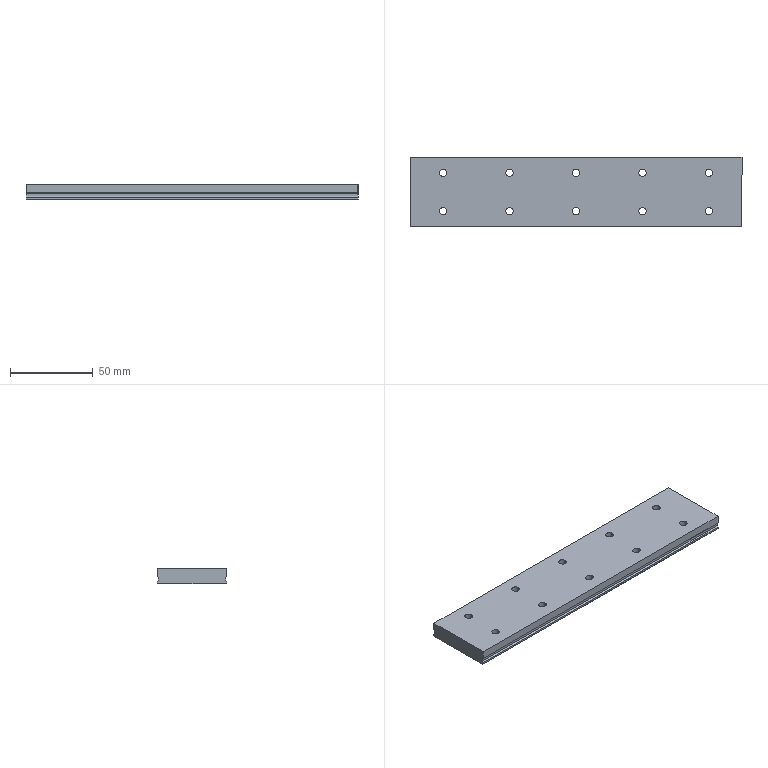Component | SolidWorks | SRS15WM-240GuideRail-2-2 | 1 solid | 66 faces | box 200 x 42 x 9.5 mm | volume 76129 mm3 | cylinder 40 | plane 26 | commonest cylinder face diameters 4.5 x20 8 x20
build123d program:
from build123d import *

# Parameters (mm, degrees)
BOSS_EXTRUDE1_DEPTH                                 = 200
CHAMFER1_SIZE                                       = 0.5
M4_COUNTERSUNK_HOLE_FOR_SOCKET_HEAD_CAP_D           = 4.5
M4_COUNTERSUNK_HOLE_FOR_SOCKET_HEAD_CAP_CBORE_D     = 8
M4_COUNTERSUNK_HOLE_FOR_SOCKET_HEAD_CAP_CBORE_DEPTH = 4
LPATTERN1_COUNT                                     = 5
LPATTERN1_PITCH                                     = 40


with BuildPart() as part:
    # Sketch1 → Boss-Extrude1 (new body)
    with BuildSketch(Plane.XY):
        Polygon((0, 8), (0.8, 7.2), (0.8, 5.7), (0, 4.9), (0, 0), (42, 0), (42, 4.9), (41.2, 5.7), (41.2, 7.2), (42, 8), (42, 9.5), (0, 9.5), align=None)
    extrude(amount=BOSS_EXTRUDE1_DEPTH)

    # Chamfer1
    chamfer1_edges = [part.edges().sort_by_distance(p)[0] for p in [
        (0, 9.5, 100),
        (42, 9.5, 100),
    ]]
    chamfer(chamfer1_edges, length=CHAMFER1_SIZE)

    # M4 Countersunk Hole for Socket Head Cap (through all)
    with Locations(Plane(origin=(0, 9.5, 0), x_dir=(1, 0, 0), z_dir=(0, 1, 0))):
        with Locations((9.5, -20), (32.5, -20)):
            m4_countersunk_hole_for_socket_head_cap = CounterBoreHole(M4_COUNTERSUNK_HOLE_FOR_SOCKET_HEAD_CAP_D / 2, M4_COUNTERSUNK_HOLE_FOR_SOCKET_HEAD_CAP_CBORE_D / 2, M4_COUNTERSUNK_HOLE_FOR_SOCKET_HEAD_CAP_CBORE_DEPTH)

    # LPattern1: M4 Countersunk Hole for Socket Head Cap ×5
    with Locations(*[(0, 0, i * LPATTERN1_PITCH) for i in range(1, LPATTERN1_COUNT)]):
        add(m4_countersunk_hole_for_socket_head_cap, mode=Mode.SUBTRACT)


solid = part.part

# Placed as in the assembly
solid = solid.moved(Location((-181.522, 40.945, 36.551), (-90, 90, 0)))